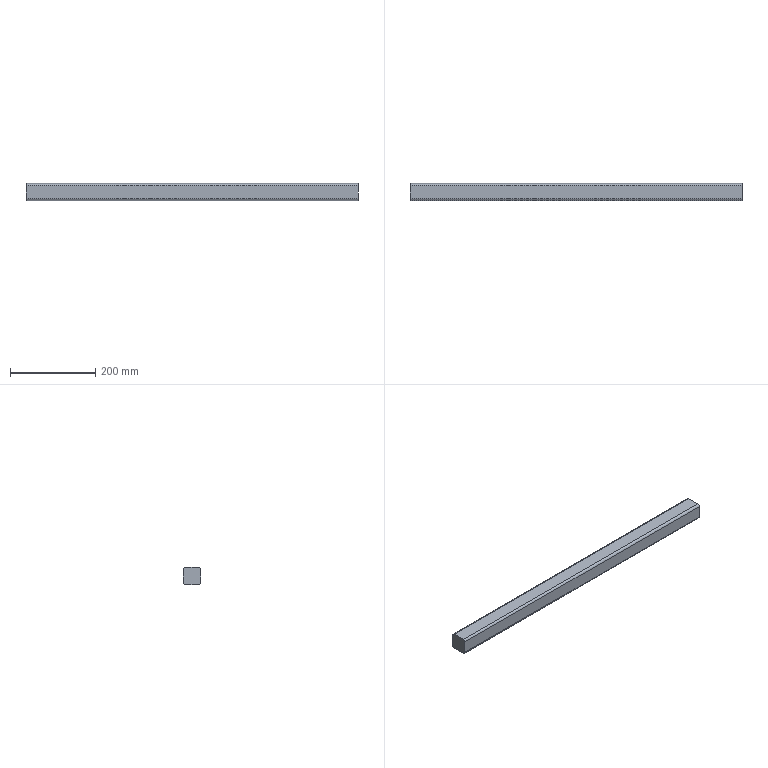Component | SolidWorks | Jig4040-780-3 | 1 solid | 10 faces | box 780 x 40 x 40 mm | volume 1231261 mm3 | plane 6 | cylinder 4 | commonest cylinder face diameters 10 x4 | material Copper
build123d program:
from build123d import *

# Parameters (mm, degrees)
BOSS_EXTRUDE1_DEPTH = 780


with BuildPart() as part:
    # Sketch1 → Boss-Extrude1 (new body)
    with BuildSketch(Plane.XY):
        with BuildLine():
            Line((5, 0), (35, 0))
            ThreePointArc((35, 0), (38.536, 1.464), (40, 5))
            Line((40, 5), (40, 35))
            ThreePointArc((40, 35), (38.536, 38.536), (35, 40))
            Line((35, 40), (5, 40))
            ThreePointArc((5, 40), (1.464, 38.536), (0, 35))
            Line((0, 35), (0, 5))
            ThreePointArc((0, 5), (1.464, 1.464), (5, 0))
        make_face()
    extrude(amount=BOSS_EXTRUDE1_DEPTH)


solid = part.part

# Placed as in the assembly
solid = solid.moved(Location((-28.008, -107.909, 1830), (0, 90, 0)))
STEP:
#1=COLOUR_RGB('',0.7922,0.8196,0.9333);
#2=FILL_AREA_STYLE_COLOUR('',#1);
#3=FILL_AREA_STYLE('',(#2));
#4=SURFACE_STYLE_FILL_AREA(#3);
#5=SURFACE_SIDE_STYLE('',(#4));
#6=SURFACE_STYLE_USAGE(.BOTH.,#5);
#7=PRESENTATION_STYLE_ASSIGNMENT((#6));
#8=CARTESIAN_POINT('',(-1.103,-4.052,72.047));
#9=VERTEX_POINT('',#8);
#10=CARTESIAN_POINT('',(-1.103,-4.248,71.85));
#11=VERTEX_POINT('',#10);
#12=CARTESIAN_POINT('',(-1.103,-4.052,71.85));
#13=DIRECTION('',(1.,0.,0.));
#14=DIRECTION('',(0.,0.,-1.));
#15=AXIS2_PLACEMENT_3D('',#12,#13,#14);
#16=CIRCLE('',#15,0.1969);
#17=EDGE_CURVE('',#9,#11,#16,.T.);
#18=ORIENTED_EDGE('',*,*,#17,.T.);
#19=CARTESIAN_POINT('',(29.606,-4.248,71.85));
#20=VERTEX_POINT('',#19);
#21=CARTESIAN_POINT('',(29.606,-4.248,71.85));
#22=DIRECTION('',(-1.,0.,0.));
#23=VECTOR('',#22,39.37);
#24=LINE('',#21,#23);
#25=EDGE_CURVE('',#20,#11,#24,.T.);
#26=ORIENTED_EDGE('',*,*,#25,.F.);
#27=CARTESIAN_POINT('',(29.606,-4.052,72.047));
#28=VERTEX_POINT('',#27);
#29=CARTESIAN_POINT('',(29.606,-4.052,71.85));
#30=DIRECTION('',(1.,0.,0.));
#31=DIRECTION('',(0.,0.,-1.));
#32=AXIS2_PLACEMENT_3D('',#29,#30,#31);
#33=CIRCLE('',#32,0.1969);
#34=EDGE_CURVE('',#28,#20,#33,.T.);
#35=ORIENTED_EDGE('',*,*,#34,.F.);
#36=CARTESIAN_POINT('',(29.606,-4.052,72.047));
#37=DIRECTION('',(-1.,0.,0.));
#38=VECTOR('',#37,39.37);
#39=LINE('',#36,#38);
#40=EDGE_CURVE('',#28,#9,#39,.T.);
#41=ORIENTED_EDGE('',*,*,#40,.T.);
#42=EDGE_LOOP('',(#18,#26,#35,#41));
#43=FACE_OUTER_BOUND('',#42,.T.);
#44=CARTESIAN_POINT('',(29.606,-4.052,71.85));
#45=DIRECTION('',(-1.,0.,0.));
#46=DIRECTION('',(0.,0.,1.));
#47=AXIS2_PLACEMENT_3D('',#44,#45,#46);
#48=CYLINDRICAL_SURFACE('',#47,0.1969);
#49=ADVANCED_FACE('',(#43),#48,.T.);
#50=CARTESIAN_POINT('',(-1.103,-4.248,70.669));
#51=VERTEX_POINT('',#50);
#52=CARTESIAN_POINT('',(-1.103,-4.248,71.85));
#53=DIRECTION('',(0.,0.,-1.));
#54=VECTOR('',#53,39.37);
#55=LINE('',#52,#54);
#56=EDGE_CURVE('',#11,#51,#55,.T.);
#57=ORIENTED_EDGE('',*,*,#56,.T.);
#58=CARTESIAN_POINT('',(29.606,-4.248,70.669));
#59=VERTEX_POINT('',#58);
#60=CARTESIAN_POINT('',(29.606,-4.248,70.669));
#61=DIRECTION('',(-1.,0.,0.));
#62=VECTOR('',#61,39.37);
#63=LINE('',#60,#62);
#64=EDGE_CURVE('',#59,#51,#63,.T.);
#65=ORIENTED_EDGE('',*,*,#64,.F.);
#66=CARTESIAN_POINT('',(29.606,-4.248,71.85));
#67=DIRECTION('',(0.,0.,-1.));
#68=VECTOR('',#67,39.37);
#69=LINE('',#66,#68);
#70=EDGE_CURVE('',#20,#59,#69,.T.);
#71=ORIENTED_EDGE('',*,*,#70,.F.);
#72=ORIENTED_EDGE('',*,*,#25,.T.);
#73=EDGE_LOOP('',(#57,#65,#71,#72));
#74=FACE_OUTER_BOUND('',#73,.T.);
#75=CARTESIAN_POINT('',(29.606,-4.248,71.85));
#76=DIRECTION('',(0.,1.,0.));
#77=DIRECTION('',(1.,0.,0.));
#78=AXIS2_PLACEMENT_3D('',#75,#76,#77);
#79=PLANE('',#78);
#80=ADVANCED_FACE('',(#74),#79,.F.);
#81=CARTESIAN_POINT('',(-1.103,-4.052,70.472));
#82=VERTEX_POINT('',#81);
#83=CARTESIAN_POINT('',(-1.103,-4.052,70.669));
#84=DIRECTION('',(1.,0.,0.));
#85=DIRECTION('',(0.,0.,-1.));
#86=AXIS2_PLACEMENT_3D('',#83,#84,#85);
#87=CIRCLE('',#86,0.1969);
#88=EDGE_CURVE('',#51,#82,#87,.T.);
#89=ORIENTED_EDGE('',*,*,#88,.T.);
#90=CARTESIAN_POINT('',(29.606,-4.052,70.472));
#91=VERTEX_POINT('',#90);
#92=CARTESIAN_POINT('',(29.606,-4.052,70.472));
#93=DIRECTION('',(-1.,0.,0.));
#94=VECTOR('',#93,39.37);
#95=LINE('',#92,#94);
#96=EDGE_CURVE('',#91,#82,#95,.T.);
#97=ORIENTED_EDGE('',*,*,#96,.F.);
#98=CARTESIAN_POINT('',(29.606,-4.052,70.669));
#99=DIRECTION('',(1.,0.,0.));
#100=DIRECTION('',(0.,0.,-1.));
#101=AXIS2_PLACEMENT_3D('',#98,#99,#100);
#102=CIRCLE('',#101,0.1969);
#103=EDGE_CURVE('',#59,#91,#102,.T.);
#104=ORIENTED_EDGE('',*,*,#103,.F.);
#105=ORIENTED_EDGE('',*,*,#64,.T.);
#106=EDGE_LOOP('',(#89,#97,#104,#105));
#107=FACE_OUTER_BOUND('',#106,.T.);
#108=CARTESIAN_POINT('',(29.606,-4.052,70.669));
#109=DIRECTION('',(-1.,0.,0.));
#110=DIRECTION('',(0.,0.,1.));
#111=AXIS2_PLACEMENT_3D('',#108,#109,#110);
#112=CYLINDRICAL_SURFACE('',#111,0.1969);
#113=ADVANCED_FACE('',(#107),#112,.T.);
#114=CARTESIAN_POINT('',(-1.103,-2.87,70.472));
#115=VERTEX_POINT('',#114);
#116=CARTESIAN_POINT('',(-1.103,-4.052,70.472));
#117=DIRECTION('',(0.,1.,0.));
#118=VECTOR('',#117,39.37);
#119=LINE('',#116,#118);
#120=EDGE_CURVE('',#82,#115,#119,.T.);
#121=ORIENTED_EDGE('',*,*,#120,.T.);
#122=CARTESIAN_POINT('',(29.606,-2.87,70.472));
#123=VERTEX_POINT('',#122);
#124=CARTESIAN_POINT('',(29.606,-2.87,70.472));
#125=DIRECTION('',(-1.,0.,0.));
#126=VECTOR('',#125,39.37);
#127=LINE('',#124,#126);
#128=EDGE_CURVE('',#123,#115,#127,.T.);
#129=ORIENTED_EDGE('',*,*,#128,.F.);
#130=CARTESIAN_POINT('',(29.606,-4.052,70.472));
#131=DIRECTION('',(0.,1.,0.));
#132=VECTOR('',#131,39.37);
#133=LINE('',#130,#132);
#134=EDGE_CURVE('',#91,#123,#133,.T.);
#135=ORIENTED_EDGE('',*,*,#134,.F.);
#136=ORIENTED_EDGE('',*,*,#96,.T.);
#137=EDGE_LOOP('',(#121,#129,#135,#136));
#138=FACE_OUTER_BOUND('',#137,.T.);
#139=CARTESIAN_POINT('',(29.606,-4.052,70.472));
#140=DIRECTION('',(0.,0.,1.));
#141=DIRECTION('',(1.,0.,0.));
#142=AXIS2_PLACEMENT_3D('',#139,#140,#141);
#143=PLANE('',#142);
#144=ADVANCED_FACE('',(#138),#143,.F.);
#145=CARTESIAN_POINT('',(-1.103,-2.674,70.669));
#146=VERTEX_POINT('',#145);
#147=CARTESIAN_POINT('',(-1.103,-2.87,70.669));
#148=DIRECTION('',(1.,0.,0.));
#149=DIRECTION('',(0.,0.,-1.));
#150=AXIS2_PLACEMENT_3D('',#147,#148,#149);
#151=CIRCLE('',#150,0.1969);
#152=EDGE_CURVE('',#115,#146,#151,.T.);
#153=ORIENTED_EDGE('',*,*,#152,.T.);
#154=CARTESIAN_POINT('',(29.606,-2.674,70.669));
#155=VERTEX_POINT('',#154);
#156=CARTESIAN_POINT('',(29.606,-2.674,70.669));
#157=DIRECTION('',(-1.,0.,0.));
#158=VECTOR('',#157,39.37);
#159=LINE('',#156,#158);
#160=EDGE_CURVE('',#155,#146,#159,.T.);
#161=ORIENTED_EDGE('',*,*,#160,.F.);
#162=CARTESIAN_POINT('',(29.606,-2.87,70.669));
#163=DIRECTION('',(1.,0.,0.));
#164=DIRECTION('',(0.,0.,-1.));
#165=AXIS2_PLACEMENT_3D('',#162,#163,#164);
#166=CIRCLE('',#165,0.1969);
#167=EDGE_CURVE('',#123,#155,#166,.T.);
#168=ORIENTED_EDGE('',*,*,#167,.F.);
#169=ORIENTED_EDGE('',*,*,#128,.T.);
#170=EDGE_LOOP('',(#153,#161,#168,#169));
#171=FACE_OUTER_BOUND('',#170,.T.);
#172=CARTESIAN_POINT('',(29.606,-2.87,70.669));
#173=DIRECTION('',(-1.,0.,0.));
#174=DIRECTION('',(0.,0.,1.));
#175=AXIS2_PLACEMENT_3D('',#172,#173,#174);
#176=CYLINDRICAL_SURFACE('',#175,0.1969);
#177=ADVANCED_FACE('',(#171),#176,.T.);
#178=CARTESIAN_POINT('',(-1.103,-2.674,71.85));
#179=VERTEX_POINT('',#178);
#180=CARTESIAN_POINT('',(-1.103,-2.674,71.85));
#181=DIRECTION('',(0.,0.,1.));
#182=VECTOR('',#181,39.37);
#183=LINE('',#180,#182);
#184=EDGE_CURVE('',#146,#179,#183,.T.);
#185=ORIENTED_EDGE('',*,*,#184,.T.);
#186=CARTESIAN_POINT('',(29.606,-2.674,71.85));
#187=VERTEX_POINT('',#186);
#188=CARTESIAN_POINT('',(29.606,-2.674,71.85));
#189=DIRECTION('',(-1.,0.,0.));
#190=VECTOR('',#189,39.37);
#191=LINE('',#188,#190);
#192=EDGE_CURVE('',#187,#179,#191,.T.);
#193=ORIENTED_EDGE('',*,*,#192,.F.);
#194=CARTESIAN_POINT('',(29.606,-2.674,71.85));
#195=DIRECTION('',(0.,0.,1.));
#196=VECTOR('',#195,39.37);
#197=LINE('',#194,#196);
#198=EDGE_CURVE('',#155,#187,#197,.T.);
#199=ORIENTED_EDGE('',*,*,#198,.F.);
#200=ORIENTED_EDGE('',*,*,#160,.T.);
#201=EDGE_LOOP('',(#185,#193,#199,#200));
#202=FACE_OUTER_BOUND('',#201,.T.);
#203=CARTESIAN_POINT('',(29.606,-2.674,71.85));
#204=DIRECTION('',(0.,-1.,0.));
#205=DIRECTION('',(-1.,0.,0.));
#206=AXIS2_PLACEMENT_3D('',#203,#204,#205);
#207=PLANE('',#206);
#208=ADVANCED_FACE('',(#202),#207,.F.);
#209=CARTESIAN_POINT('',(-1.103,-2.87,72.047));
#210=VERTEX_POINT('',#209);
#211=CARTESIAN_POINT('',(-1.103,-2.87,71.85));
#212=DIRECTION('',(1.,0.,0.));
#213=DIRECTION('',(0.,0.,1.));
#214=AXIS2_PLACEMENT_3D('',#211,#212,#213);
#215=CIRCLE('',#214,0.1969);
#216=EDGE_CURVE('',#179,#210,#215,.T.);
#217=ORIENTED_EDGE('',*,*,#216,.T.);
#218=CARTESIAN_POINT('',(29.606,-2.87,72.047));
#219=VERTEX_POINT('',#218);
#220=CARTESIAN_POINT('',(29.606,-2.87,72.047));
#221=DIRECTION('',(-1.,0.,0.));
#222=VECTOR('',#221,39.37);
#223=LINE('',#220,#222);
#224=EDGE_CURVE('',#219,#210,#223,.T.);
#225=ORIENTED_EDGE('',*,*,#224,.F.);
#226=CARTESIAN_POINT('',(29.606,-2.87,71.85));
#227=DIRECTION('',(1.,0.,0.));
#228=DIRECTION('',(0.,0.,1.));
#229=AXIS2_PLACEMENT_3D('',#226,#227,#228);
#230=CIRCLE('',#229,0.1969);
#231=EDGE_CURVE('',#187,#219,#230,.T.);
#232=ORIENTED_EDGE('',*,*,#231,.F.);
#233=ORIENTED_EDGE('',*,*,#192,.T.);
#234=EDGE_LOOP('',(#217,#225,#232,#233));
#235=FACE_OUTER_BOUND('',#234,.T.);
#236=CARTESIAN_POINT('',(29.606,-2.87,71.85));
#237=DIRECTION('',(-1.,0.,0.));
#238=DIRECTION('',(0.,0.,1.));
#239=AXIS2_PLACEMENT_3D('',#236,#237,#238);
#240=CYLINDRICAL_SURFACE('',#239,0.1969);
#241=ADVANCED_FACE('',(#235),#240,.T.);
#242=CARTESIAN_POINT('',(-1.103,-4.052,72.047));
#243=DIRECTION('',(0.,-1.,0.));
#244=VECTOR('',#243,39.37);
#245=LINE('',#242,#244);
#246=EDGE_CURVE('',#210,#9,#245,.T.);
#247=ORIENTED_EDGE('',*,*,#246,.T.);
#248=ORIENTED_EDGE('',*,*,#40,.F.);
#249=CARTESIAN_POINT('',(29.606,-4.052,72.047));
#250=DIRECTION('',(0.,-1.,0.));
#251=VECTOR('',#250,39.37);
#252=LINE('',#249,#251);
#253=EDGE_CURVE('',#219,#28,#252,.T.);
#254=ORIENTED_EDGE('',*,*,#253,.F.);
#255=ORIENTED_EDGE('',*,*,#224,.T.);
#256=EDGE_LOOP('',(#247,#248,#254,#255));
#257=FACE_OUTER_BOUND('',#256,.T.);
#258=CARTESIAN_POINT('',(29.606,-4.052,72.047));
#259=DIRECTION('',(0.,0.,-1.));
#260=DIRECTION('',(-1.,0.,0.));
#261=AXIS2_PLACEMENT_3D('',#258,#259,#260);
#262=PLANE('',#261);
#263=ADVANCED_FACE('',(#257),#262,.F.);
#264=ORIENTED_EDGE('',*,*,#34,.T.);
#265=ORIENTED_EDGE('',*,*,#70,.T.);
#266=ORIENTED_EDGE('',*,*,#103,.T.);
#267=ORIENTED_EDGE('',*,*,#134,.T.);
#268=ORIENTED_EDGE('',*,*,#167,.T.);
#269=ORIENTED_EDGE('',*,*,#198,.T.);
#270=ORIENTED_EDGE('',*,*,#231,.T.);
#271=ORIENTED_EDGE('',*,*,#253,.T.);
#272=EDGE_LOOP('',(#264,#265,#266,#267,#268,#269,#270,#271));
#273=FACE_OUTER_BOUND('',#272,.T.);
#274=CARTESIAN_POINT('',(29.606,-4.052,71.85));
#275=DIRECTION('',(1.,0.,0.));
#276=DIRECTION('',(0.,0.,-1.));
#277=AXIS2_PLACEMENT_3D('',#274,#275,#276);
#278=PLANE('',#277);
#279=ADVANCED_FACE('',(#273),#278,.T.);
#280=ORIENTED_EDGE('',*,*,#17,.F.);
#281=ORIENTED_EDGE('',*,*,#246,.F.);
#282=ORIENTED_EDGE('',*,*,#216,.F.);
#283=ORIENTED_EDGE('',*,*,#184,.F.);
#284=ORIENTED_EDGE('',*,*,#152,.F.);
#285=ORIENTED_EDGE('',*,*,#120,.F.);
#286=ORIENTED_EDGE('',*,*,#88,.F.);
#287=ORIENTED_EDGE('',*,*,#56,.F.);
#288=EDGE_LOOP('',(#280,#281,#282,#283,#284,#285,#286,#287));
#289=FACE_OUTER_BOUND('',#288,.T.);
#290=CARTESIAN_POINT('',(-1.103,-4.052,71.85));
#291=DIRECTION('',(1.,0.,0.));
#292=DIRECTION('',(0.,0.,-1.));
#293=AXIS2_PLACEMENT_3D('',#290,#291,#292);
#294=PLANE('',#293);
#295=ADVANCED_FACE('',(#289),#294,.F.);
#296=CLOSED_SHELL('',(#49,#80,#113,#144,#177,#208,#241,#263,#279,#295));
#297=MANIFOLD_SOLID_BREP('',#296);
#298=STYLED_ITEM('',(#7),#297);
#299=(LENGTH_UNIT()NAMED_UNIT(*)SI_UNIT($,.METRE.));
#300=LENGTH_MEASURE_WITH_UNIT(LENGTH_MEASURE(0.0254),#299);
#301=DIMENSIONAL_EXPONENTS(1.,0.,0.,0.,0.,0.,0.);
#302=(CONVERSION_BASED_UNIT('',#300)LENGTH_UNIT()NAMED_UNIT(#301));
#303=UNCERTAINTY_MEASURE_WITH_UNIT(LENGTH_MEASURE(0.00001),#302,'','');
#304=(NAMED_UNIT(*)PLANE_ANGLE_UNIT()SI_UNIT($,.RADIAN.));
#305=(NAMED_UNIT(*)SI_UNIT($,.STERADIAN.)SOLID_ANGLE_UNIT());
#306=(GEOMETRIC_REPRESENTATION_CONTEXT(3)GLOBAL_UNCERTAINTY_ASSIGNED_CONTEXT((#303))GLOBAL_UNIT_ASSIGNED_CONTEXT((#302,#304,#305))REPRESENTATION_CONTEXT('',''));
#307=MECHANICAL_DESIGN_GEOMETRIC_PRESENTATION_REPRESENTATION('',(#298),#306);
#308=CARTESIAN_POINT('',(0.,0.,0.));
#309=DIRECTION('',(0.,0.,1.));
#310=DIRECTION('',(1.,0.,0.));
#311=AXIS2_PLACEMENT_3D('',#308,#309,#310);
#312=(LENGTH_UNIT()NAMED_UNIT(*)SI_UNIT($,.METRE.));
#313=LENGTH_MEASURE_WITH_UNIT(LENGTH_MEASURE(0.0254),#312);
#314=DIMENSIONAL_EXPONENTS(1.,0.,0.,0.,0.,0.,0.);
#315=(CONVERSION_BASED_UNIT('',#313)LENGTH_UNIT()NAMED_UNIT(#314));
#316=UNCERTAINTY_MEASURE_WITH_UNIT(LENGTH_MEASURE(0.00001),#315,'','');
#317=(NAMED_UNIT(*)PLANE_ANGLE_UNIT()SI_UNIT($,.RADIAN.));
#318=(NAMED_UNIT(*)SI_UNIT($,.STERADIAN.)SOLID_ANGLE_UNIT());
#319=(GEOMETRIC_REPRESENTATION_CONTEXT(3)GLOBAL_UNCERTAINTY_ASSIGNED_CONTEXT((#316))GLOBAL_UNIT_ASSIGNED_CONTEXT((#315,#317,#318))REPRESENTATION_CONTEXT('',''));
#320=ADVANCED_BREP_SHAPE_REPRESENTATION('',(#297,#311),#319);
#321=PRESENTATION_LAYER_ASSIGNMENT('','',(#298));